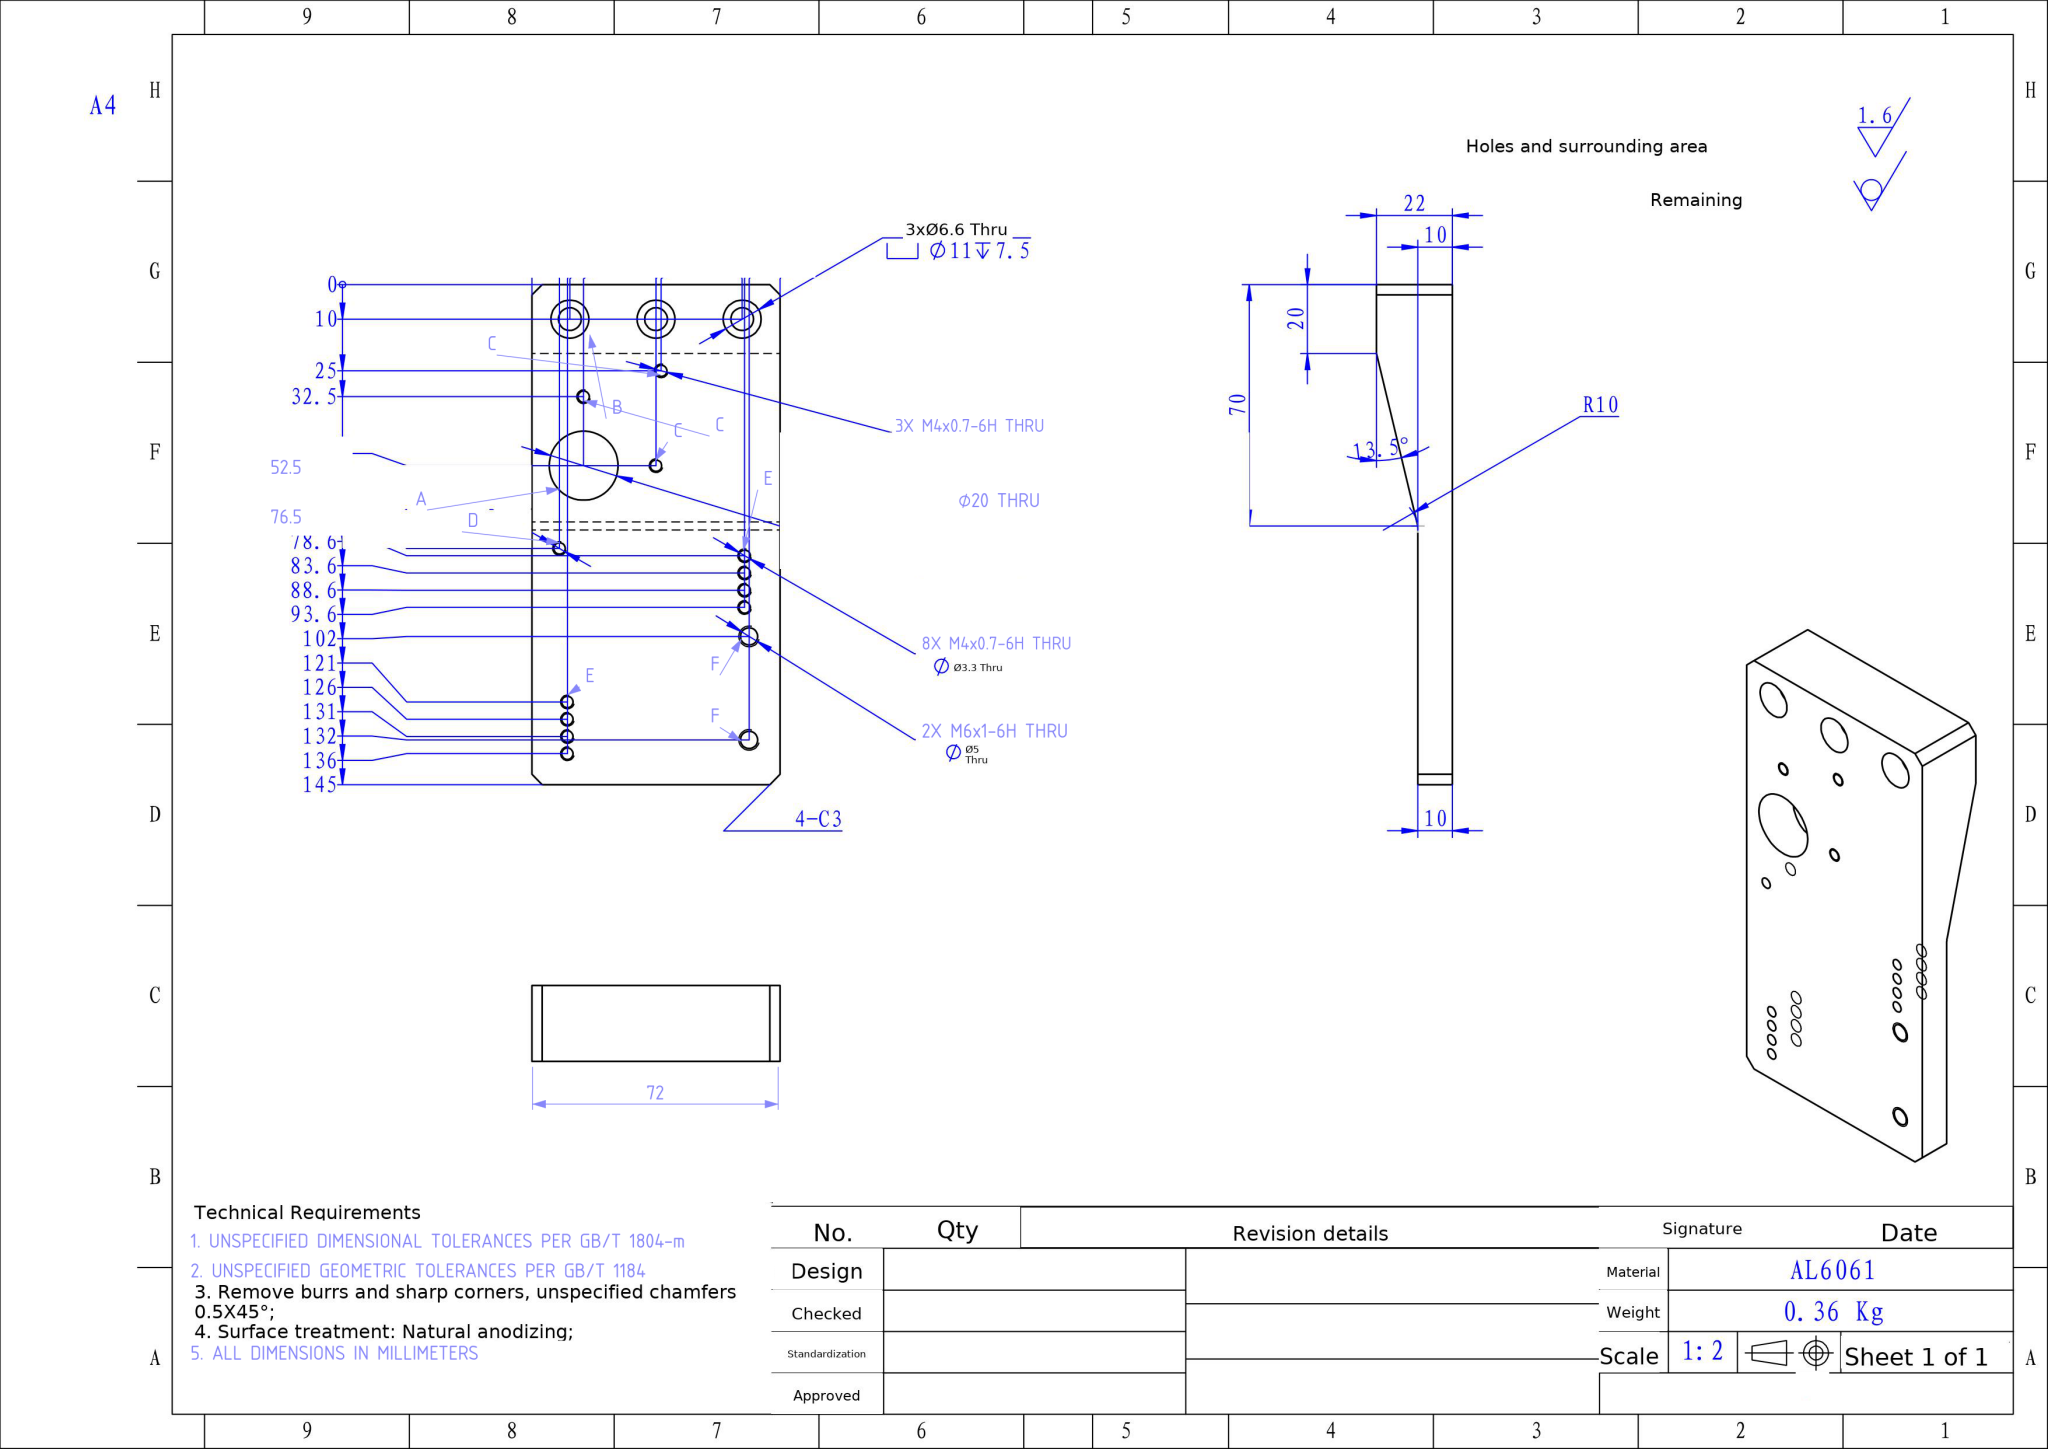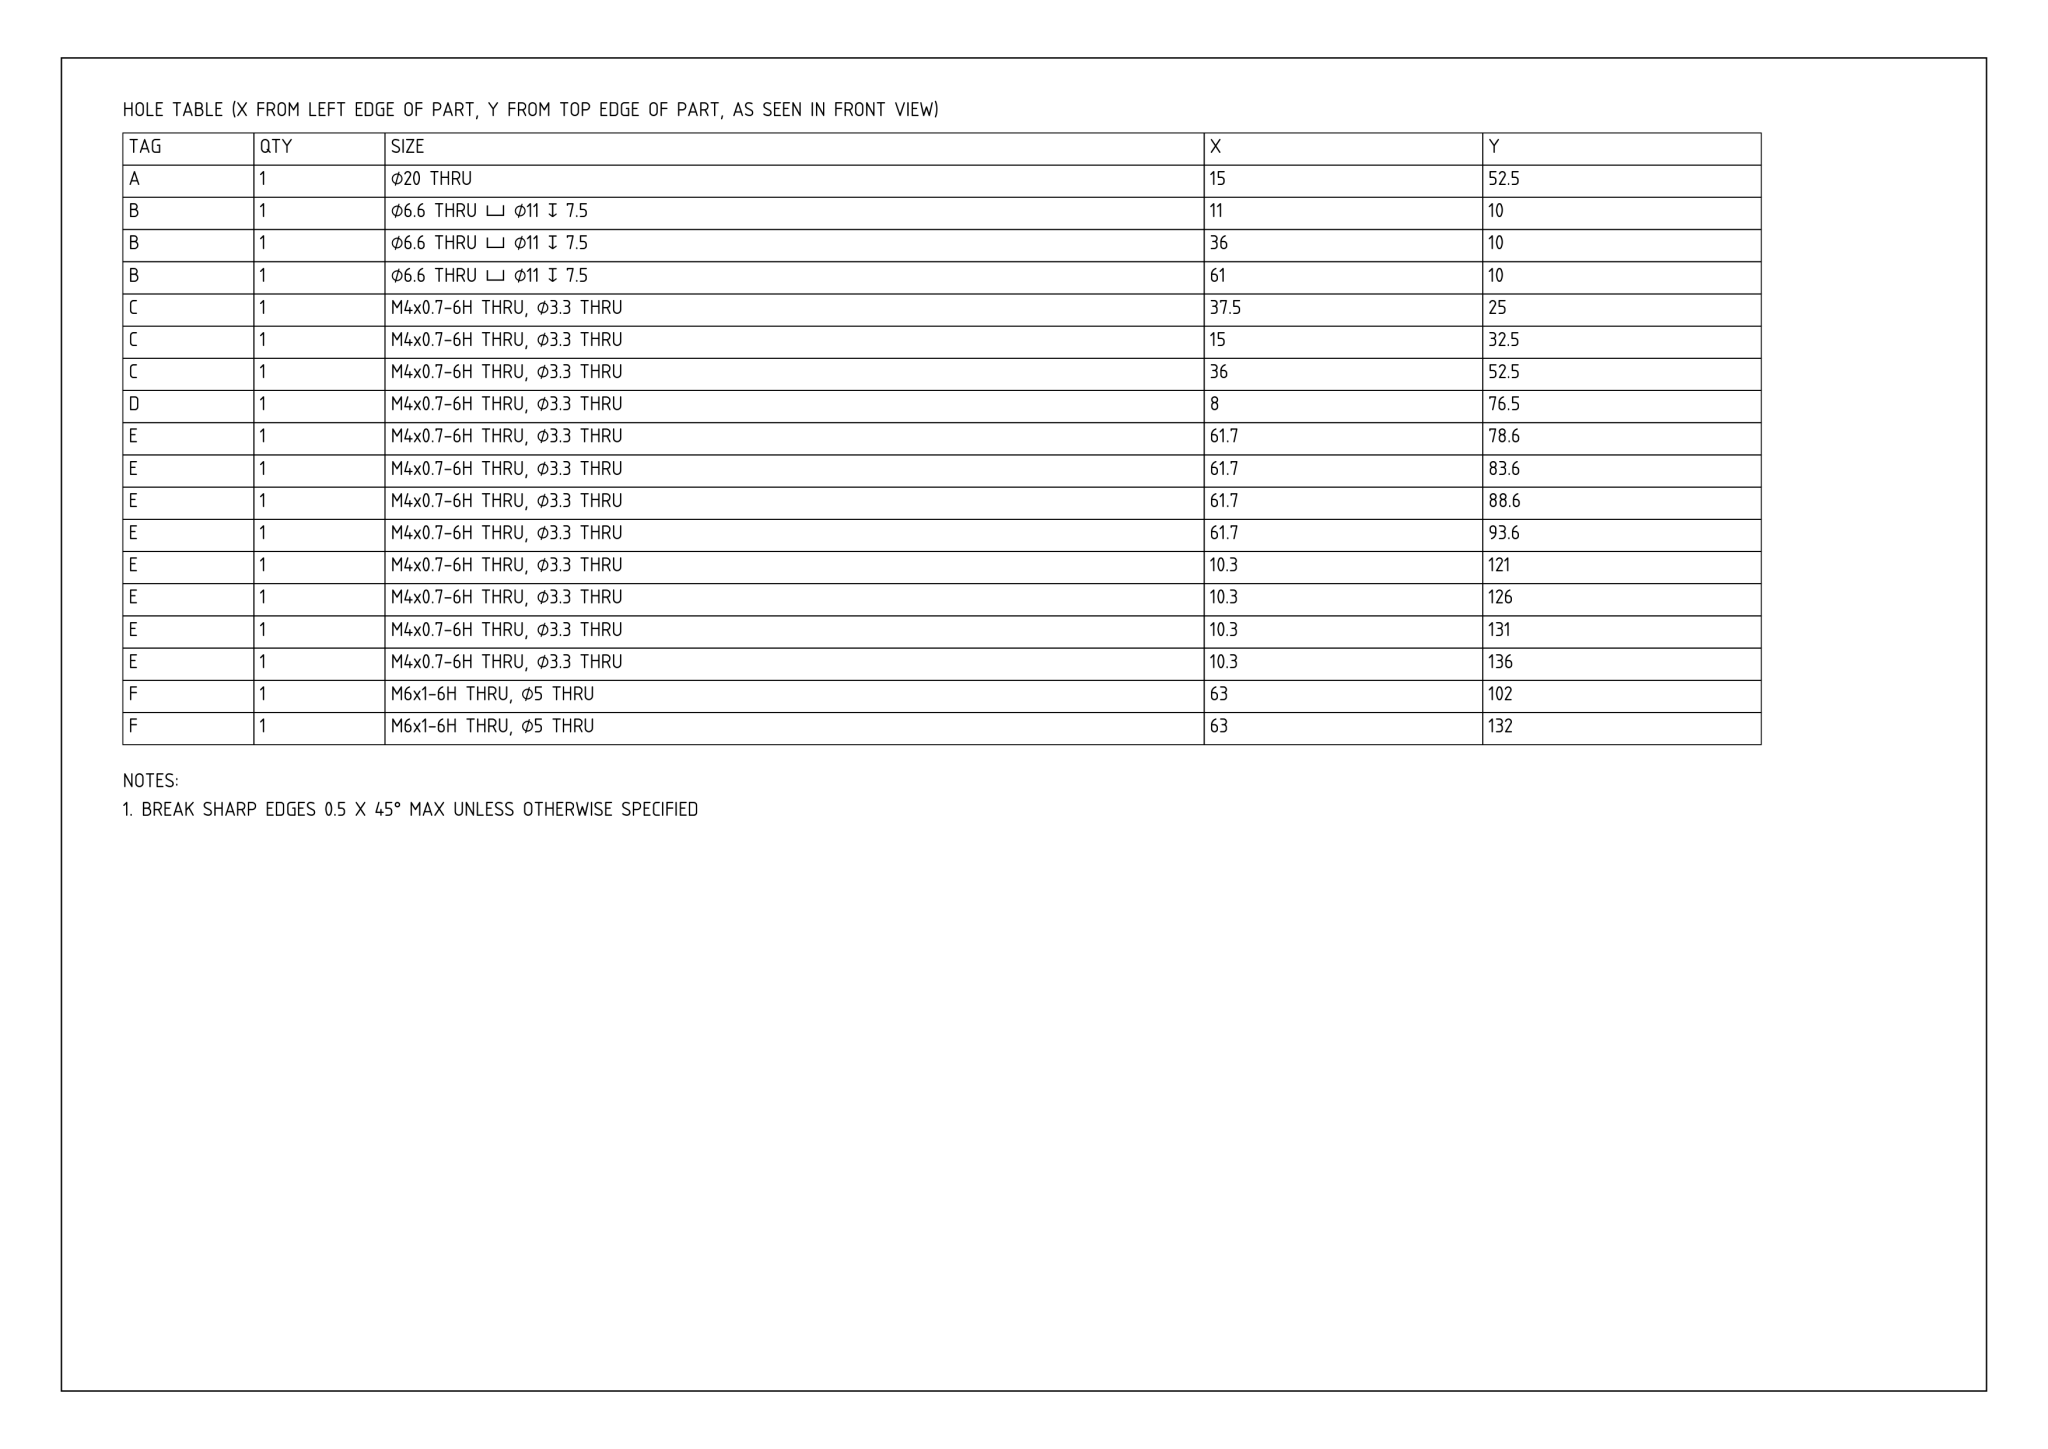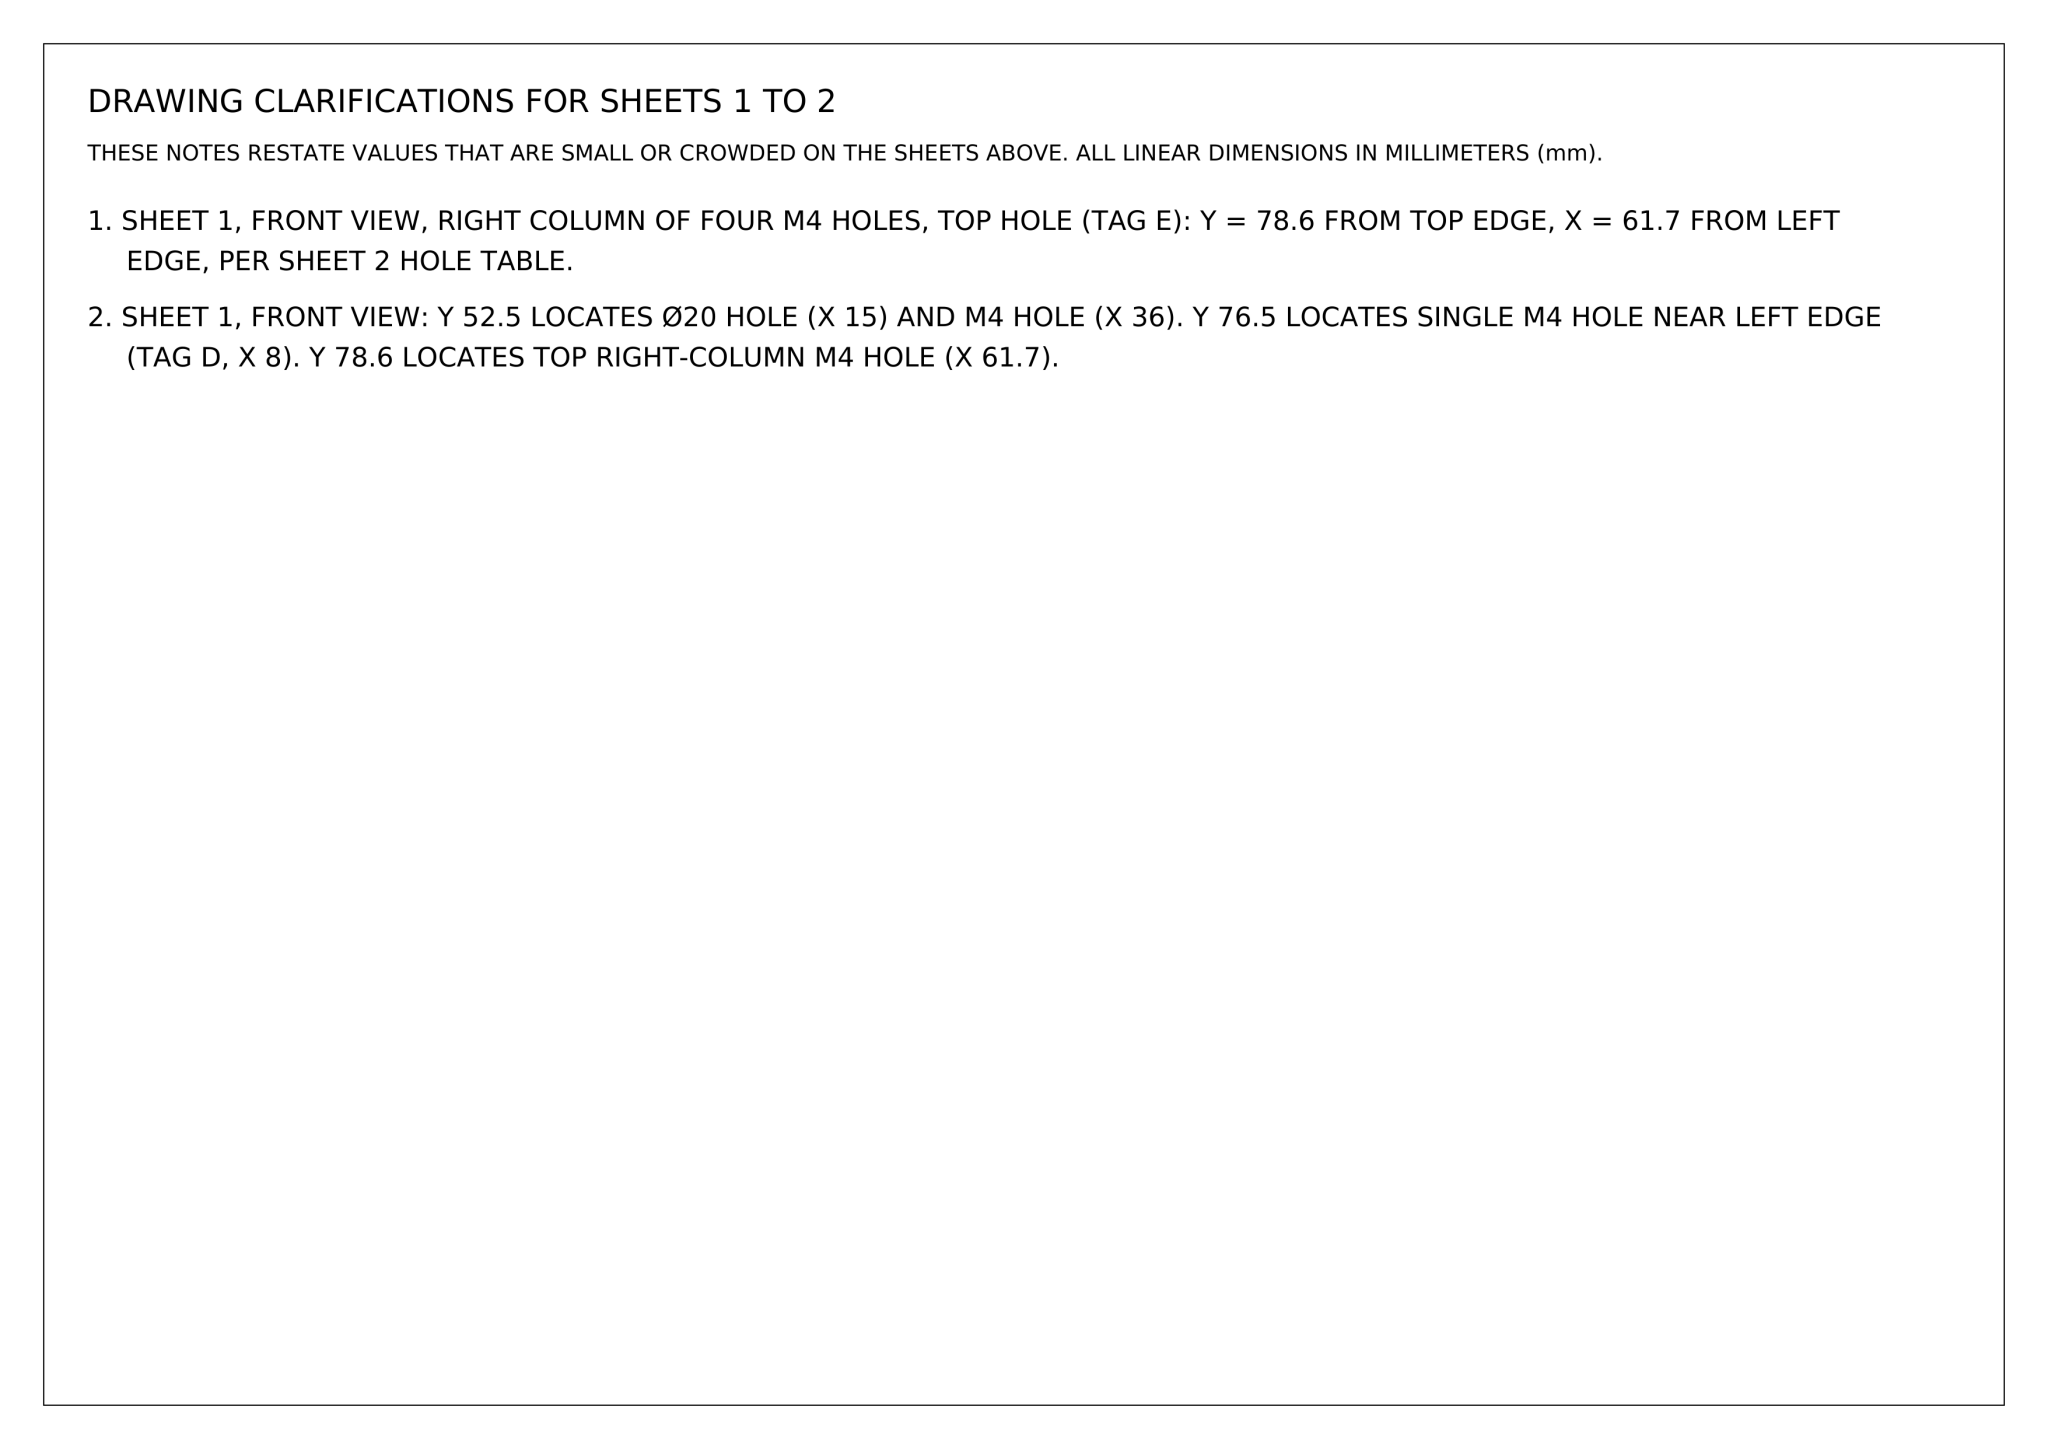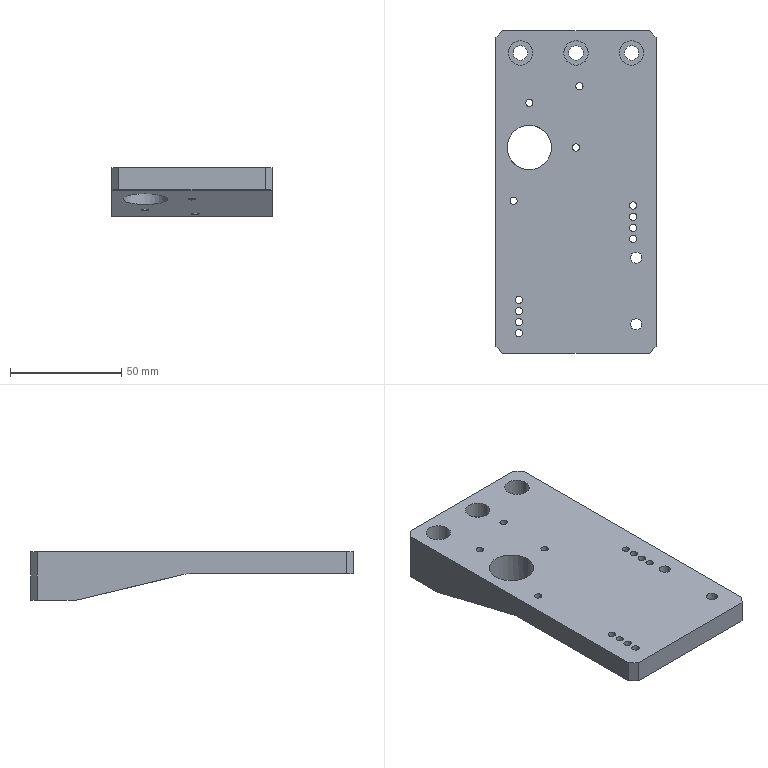Part | NX | mm | 1 solid | 58 faces | box 72 x 145 x 22 mm | volume 133284 mm3 | cylinder 43 | plane 15 | commonest cylinder face diameters 3.3 x24 11 x6 6.6 x6 5 x4 20 x3